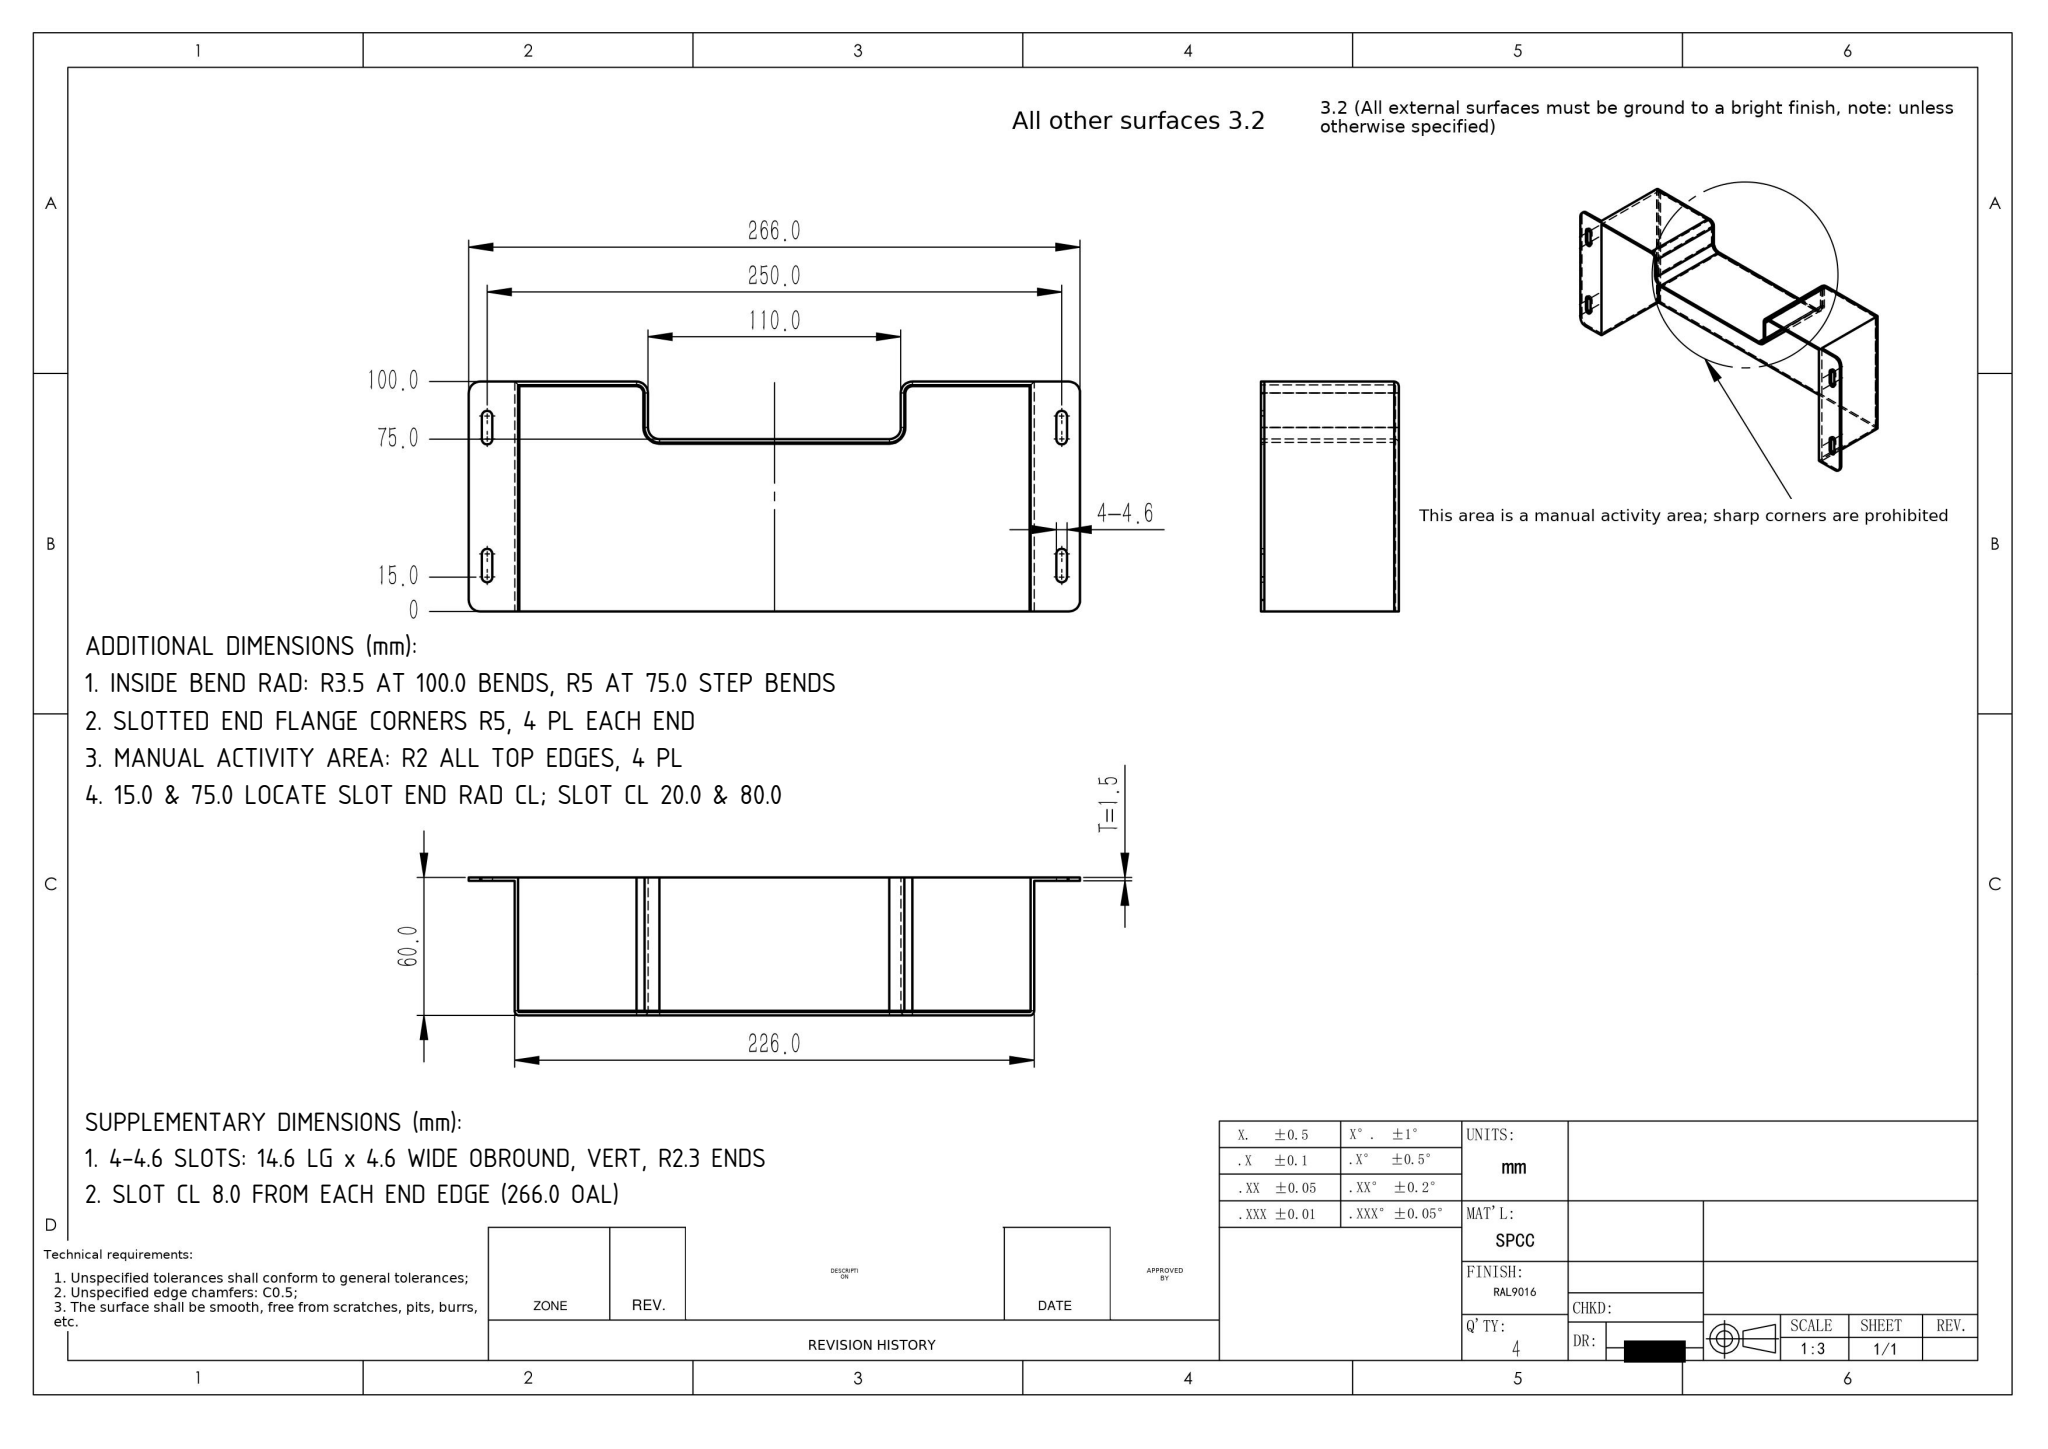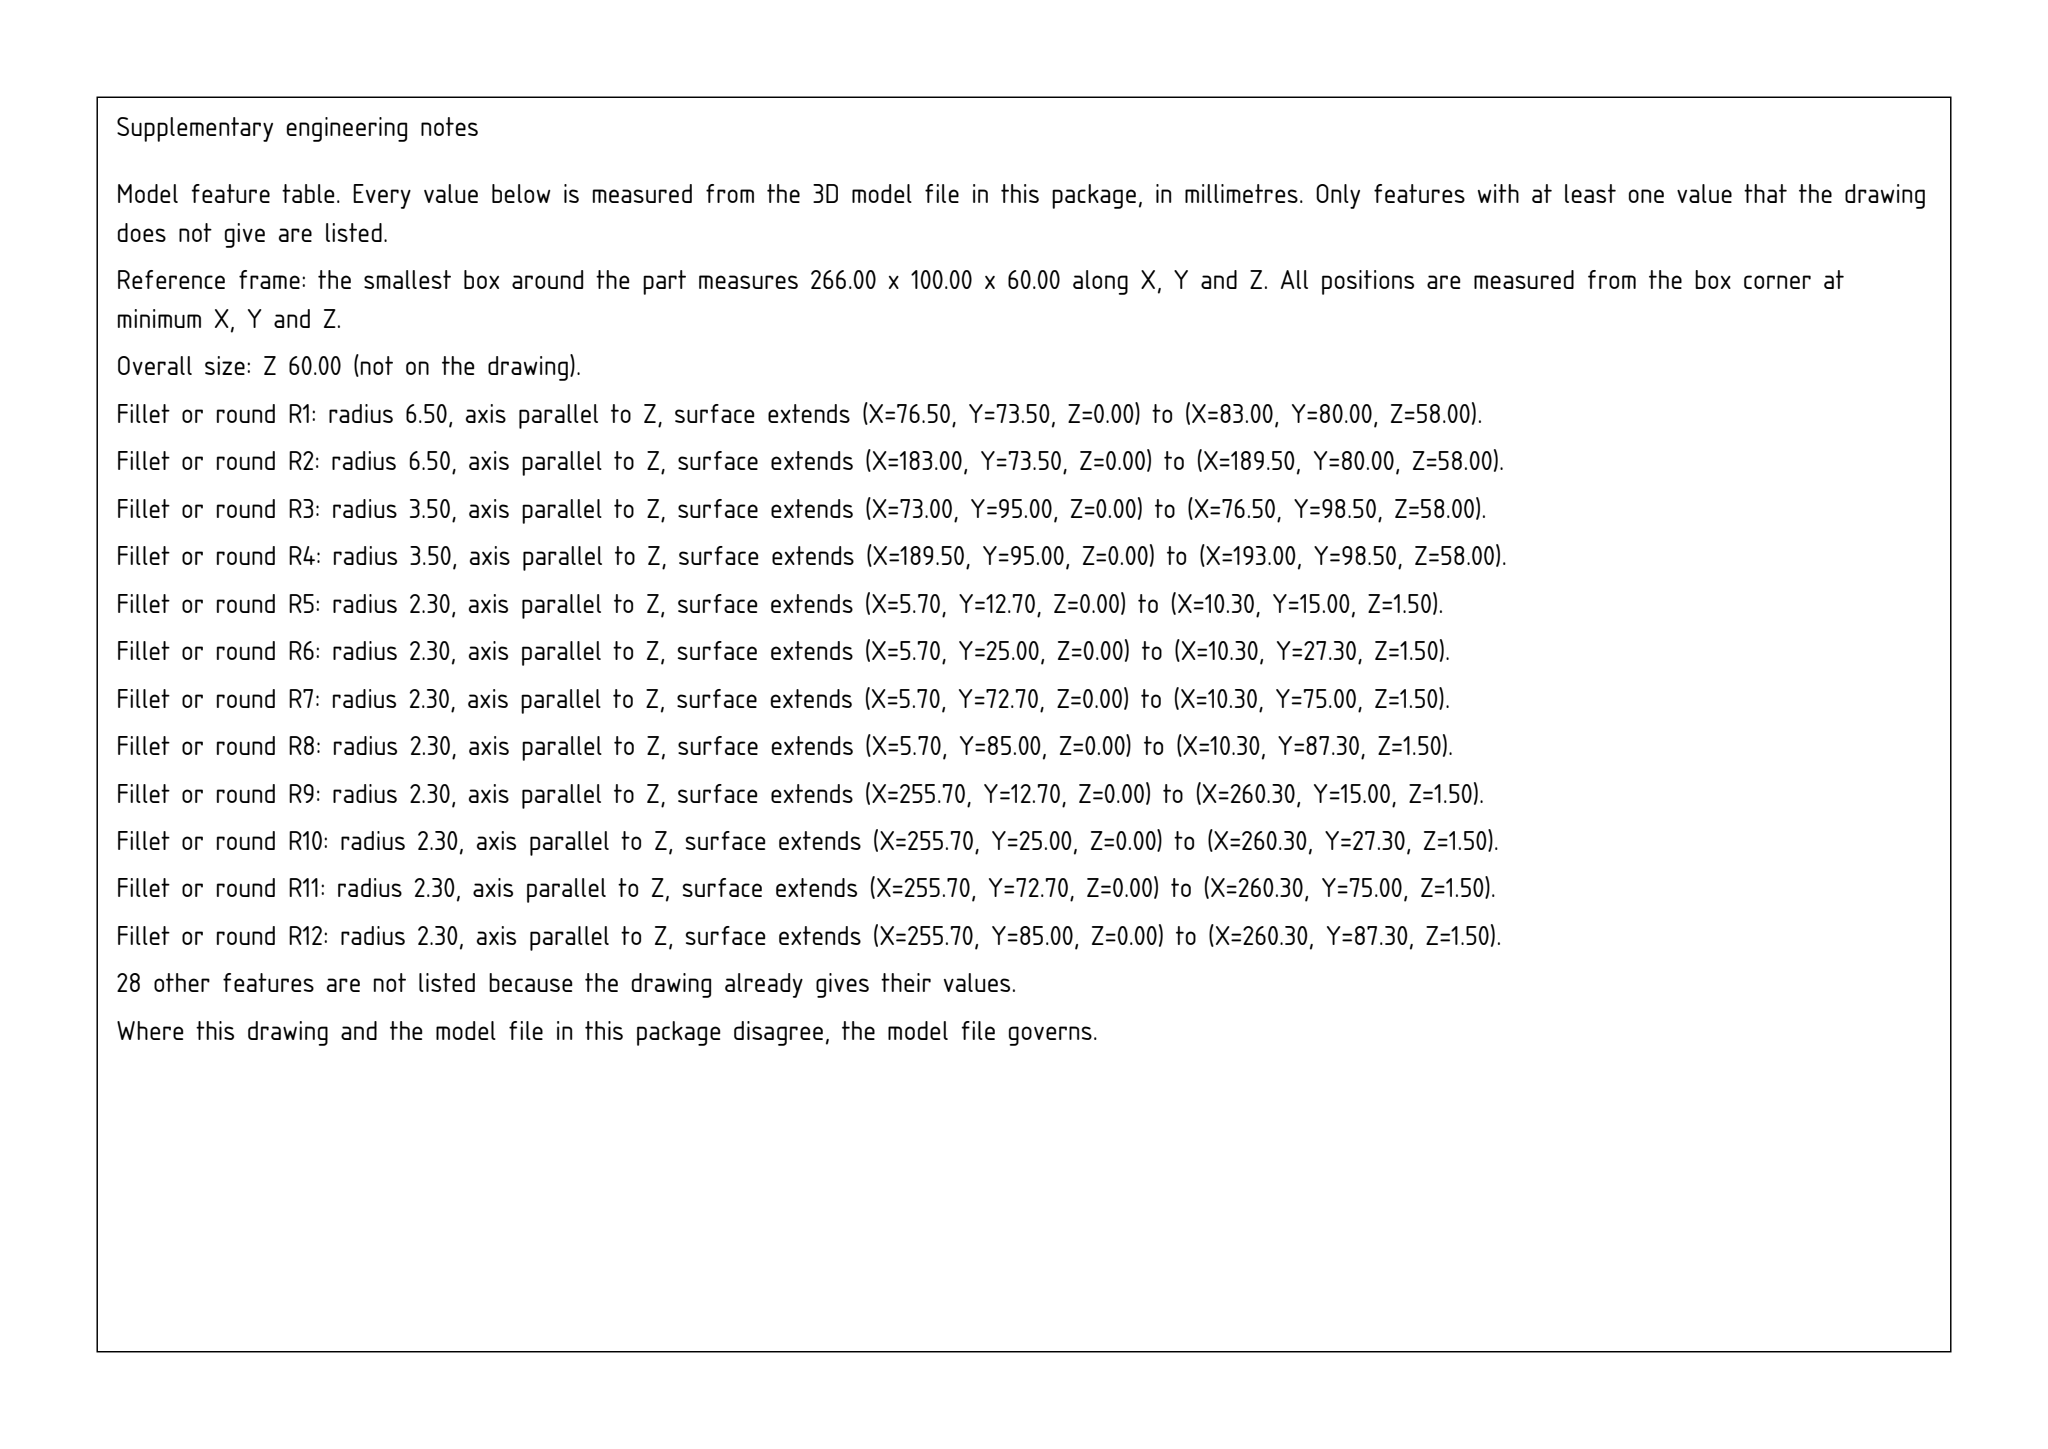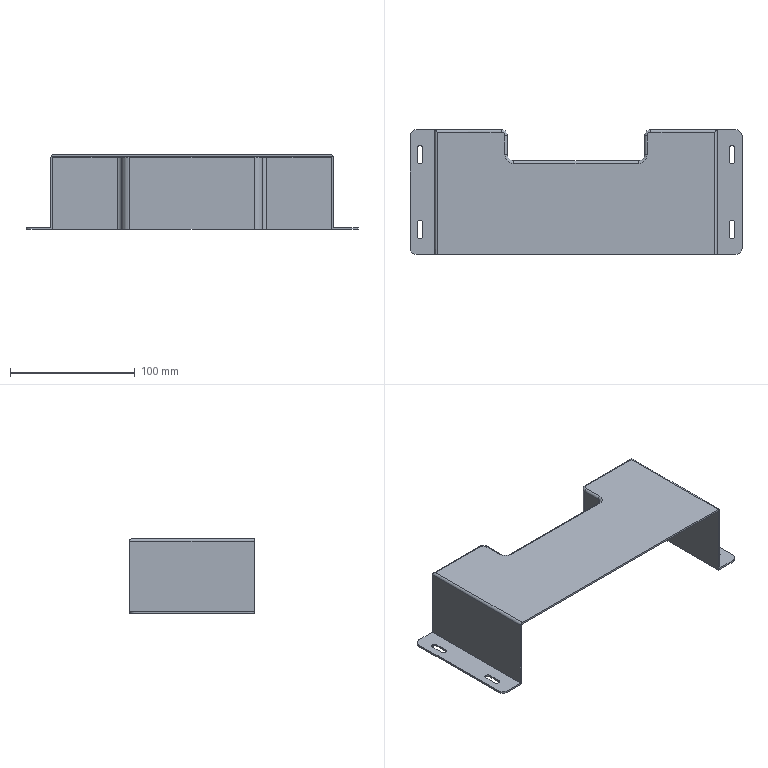Part | SolidWorks | mm | 1 solid | 72 faces | box 266 x 100 x 60 mm | volume 75745 mm3 | cylinder 34 | plane 30 | torus 8 | commonest cylinder face diameters 10 x8 4.6 x8 4 x7 1 x7 7 x2 13 x2
build123d program:
from build123d import *

# Parameters (mm, degrees)
SKETCH1_W           = 226
SKETCH1_H           = 100
BOSS_EXTRUDE1_DEPTH = 60
SKETCH2_W           = 110
SKETCH2_H           = 25
CUT_EXTRUDE2_DEPTH  = 163.385
FILLET1_R           = 5
FILLET2_R           = 2
SHELL1_T            = -1.5
SKETCH3_W           = 1.5
SKETCH3_H           = 100
BOSS_EXTRUDE2_DEPTH = 20
SKETCH4_W           = 1.5
SKETCH4_H           = 100
BOSS_EXTRUDE3_DEPTH = 20
CUT_EXTRUDE3_DEPTH  = 177.043
CUT_EXTRUDE4_REACH  = 178.887
FILLET3_R           = 5


with BuildPart() as part:
    # Sketch1 → Boss-Extrude1 (new body)
    with BuildSketch(Plane.XY):
        with Locations((0, 50)):
            Rectangle(SKETCH1_W, SKETCH1_H)
    extrude(amount=BOSS_EXTRUDE1_DEPTH)

    # Sketch2 → Cut-Extrude2 (cut, through all)
    with BuildSketch(Plane.XY.offset(60)):
        with Locations((0, 87.5)):
            Rectangle(SKETCH2_W, SKETCH2_H)
    extrude(amount=-CUT_EXTRUDE2_DEPTH, mode=Mode.SUBTRACT)

    # Fillet1
    fillet1_edges = [part.edges().sort_by_distance(p)[0] for p in [
        (-55, 75, 30),
        (-55, 100, 30),
        (55, 100, 30),
        (55, 75, 30),
    ]]
    fillet(fillet1_edges, radius=FILLET1_R)

    # Fillet2
    fillet2_edges = [part.edges().sort_by_distance(p)[0] for p in [
        (113, 50, 60),
        (86.5, 100, 60),
        (0, 75, 60),
        (-55, 87.5, 60),
        (-86.5, 100, 60),
        (55, 87.5, 60),
        (-56.464, 98.536, 60),
        (56.464, 98.536, 60),
        (-113, 50, 60),
        (53.536, 76.464, 60),
        (-53.536, 76.464, 60),
    ]]
    fillet(fillet2_edges, radius=FILLET2_R)

    # Shell1
    shell1_openings = [part.faces().sort_by_distance(p)[0] for p in [
        (0, 44.792, 0),
    ]]
    offset(amount=SHELL1_T, openings=shell1_openings)

    # Sketch3 → Boss-Extrude2 (add)
    with BuildSketch(Plane.ZY.offset(113)):
        with Locations((0.75, 50)):
            Rectangle(SKETCH3_W, SKETCH3_H)
    extrude(amount=BOSS_EXTRUDE2_DEPTH)

    # Sketch4 → Boss-Extrude3 (add)
    with BuildSketch(Plane(origin=(113, 0, 0), x_dir=(0, 0, -1), z_dir=(1, 0, 0))):
        with Locations((-0.75, 50)):
            Rectangle(SKETCH4_W, SKETCH4_H)
    extrude(amount=BOSS_EXTRUDE3_DEPTH)

    # Sketch5 → Cut-Extrude3 (cut, through all)
    with BuildSketch(Plane(origin=(0, 1.5, 0), x_dir=(1, 0, 0), z_dir=(0, 1, 0))):
        with BuildLine():
            Line((111.5, 0), (-111.5, 0))
            Line((-111.5, 0), (-111.5, -58))
            ThreePointArc((-111.5, -58), (-111.354, -58.354), (-111, -58.5))
            Line((-111, -58.5), (111, -58.5))
            ThreePointArc((111, -58.5), (111.354, -58.354), (111.5, -58))
            Line((111.5, -58), (111.5, 0))
        make_face()
    extrude(amount=-CUT_EXTRUDE3_DEPTH, mode=Mode.SUBTRACT)

    # Sketch8 → Cut-Extrude4 (cut, up to next)
    with BuildSketch(Plane(origin=(0, 0, 0), x_dir=(-1, 0, 0), z_dir=(0, 0, -1)), mode=Mode.PRIVATE) as cut_extrude4_sk1:
        with BuildLine():
            Line((-122.7, 85), (-122.7, 75))
            ThreePointArc((-122.7, 75), (-125, 72.7), (-127.3, 75))
            Line((-127.3, 75), (-127.3, 85))
            ThreePointArc((-127.3, 85), (-125, 87.3), (-122.7, 85))
        make_face()
    cut_extrude4_tool1 = extrude(cut_extrude4_sk1.sketch, amount=-CUT_EXTRUDE4_REACH, mode=Mode.PRIVATE) & part.part
    # Sketch8 → Cut-Extrude4 (cut, up to next)
    with BuildSketch(Plane(origin=(0, 0, 0), x_dir=(-1, 0, 0), z_dir=(0, 0, -1)), mode=Mode.PRIVATE) as cut_extrude4_sk2:
        with BuildLine():
            Line((-122.7, 15), (-122.7, 25))
            ThreePointArc((-122.7, 25), (-125, 27.3), (-127.3, 25))
            Line((-127.3, 25), (-127.3, 15))
            ThreePointArc((-127.3, 15), (-125, 12.7), (-122.7, 15))
        make_face()
    cut_extrude4_tool2 = extrude(cut_extrude4_sk2.sketch, amount=-CUT_EXTRUDE4_REACH, mode=Mode.PRIVATE) & part.part
    # Sketch8 → Cut-Extrude4 (cut, up to next)
    with BuildSketch(Plane(origin=(0, 0, 0), x_dir=(-1, 0, 0), z_dir=(0, 0, -1)), mode=Mode.PRIVATE) as cut_extrude4_sk3:
        with BuildLine():
            Line((122.7, 15), (122.7, 25))
            ThreePointArc((122.7, 25), (125, 27.3), (127.3, 25))
            Line((127.3, 25), (127.3, 15))
            ThreePointArc((127.3, 15), (125, 12.7), (122.7, 15))
        make_face()
    cut_extrude4_tool3 = extrude(cut_extrude4_sk3.sketch, amount=-CUT_EXTRUDE4_REACH, mode=Mode.PRIVATE) & part.part
    # Sketch8 → Cut-Extrude4 (cut, up to next)
    with BuildSketch(Plane(origin=(0, 0, 0), x_dir=(-1, 0, 0), z_dir=(0, 0, -1)), mode=Mode.PRIVATE) as cut_extrude4_sk4:
        with BuildLine():
            Line((122.7, 85), (122.7, 75))
            ThreePointArc((122.7, 75), (125, 72.7), (127.3, 75))
            Line((127.3, 75), (127.3, 85))
            ThreePointArc((127.3, 85), (125, 87.3), (122.7, 85))
        make_face()
    cut_extrude4_tool4 = extrude(cut_extrude4_sk4.sketch, amount=-CUT_EXTRUDE4_REACH, mode=Mode.PRIVATE) & part.part
    add(cut_extrude4_tool1.solids().sort_by_distance((125, 80, 0))[0], mode=Mode.SUBTRACT)
    add(cut_extrude4_tool2.solids().sort_by_distance((125, 20, 0))[0], mode=Mode.SUBTRACT)
    add(cut_extrude4_tool3.solids().sort_by_distance((-125, 20, 0))[0], mode=Mode.SUBTRACT)
    add(cut_extrude4_tool4.solids().sort_by_distance((-125, 80, 0))[0], mode=Mode.SUBTRACT)

    # Fillet3
    fillet3_edges = [part.edges().sort_by_distance(p)[0] for p in [
        (-133, 0, 0.75),
        (-133, 100, 0.75),
        (133, 100, 0.75),
        (133, 0, 0.75),
    ]]
    fillet(fillet3_edges, radius=FILLET3_R)


solid = part.part